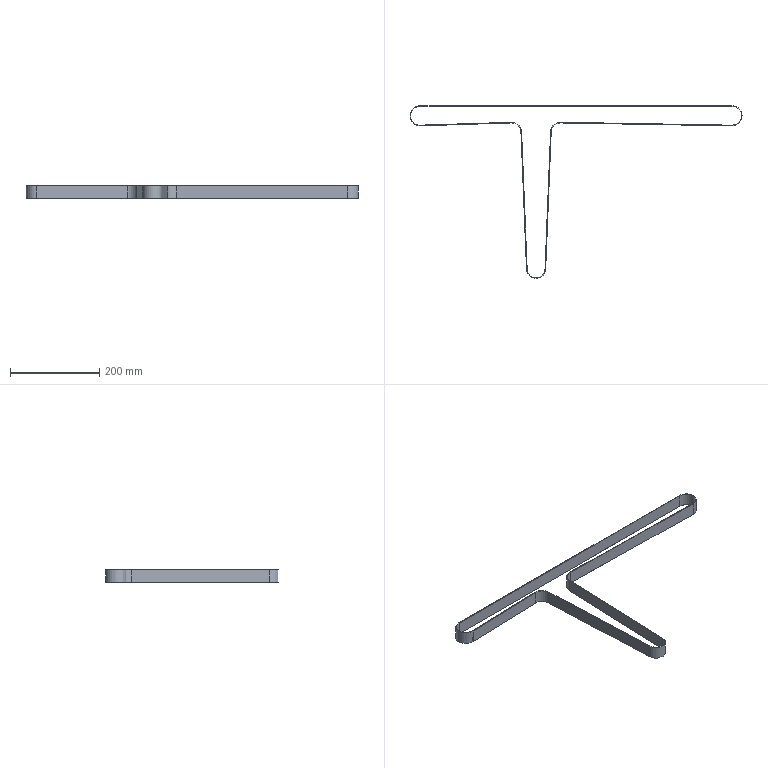Component | SolidWorks | Belt4-15^SW-111-1 | 1 solid | 24 faces | box 745 x 387 x 29 mm | volume 94519 mm3 | cylinder 12 | plane 12 | commonest cylinder face diameters 42 x5 45 x5 43 x1 40 x1
STEP:
#1=COLOUR_RGB('',0.7922,0.8196,0.9333);
#2=FILL_AREA_STYLE_COLOUR('',#1);
#3=FILL_AREA_STYLE('',(#2));
#4=SURFACE_STYLE_FILL_AREA(#3);
#5=SURFACE_SIDE_STYLE('',(#4));
#6=SURFACE_STYLE_USAGE(.BOTH.,#5);
#7=PRESENTATION_STYLE_ASSIGNMENT((#6));
#8=CARTESIAN_POINT('',(37.806,4.267,-1.437));
#9=VERTEX_POINT('',#8);
#10=CARTESIAN_POINT('',(36.98,5.094,-1.437));
#11=VERTEX_POINT('',#10);
#12=CARTESIAN_POINT('',(36.98,4.267,-1.437));
#13=DIRECTION('',(0.,0.,1.));
#14=DIRECTION('',(-1.,0.,0.));
#15=AXIS2_PLACEMENT_3D('',#12,#13,#14);
#16=CIRCLE('',#15,0.8268);
#17=EDGE_CURVE('',#9,#11,#16,.T.);
#18=ORIENTED_EDGE('',*,*,#17,.F.);
#19=CARTESIAN_POINT('',(37.806,4.267,-0.2953));
#20=VERTEX_POINT('',#19);
#21=CARTESIAN_POINT('',(37.806,4.267,-1.437));
#22=DIRECTION('',(0.,0.,1.));
#23=VECTOR('',#22,39.37);
#24=LINE('',#21,#23);
#25=EDGE_CURVE('',#9,#20,#24,.T.);
#26=ORIENTED_EDGE('',*,*,#25,.T.);
#27=CARTESIAN_POINT('',(36.98,5.094,-0.2953));
#28=VERTEX_POINT('',#27);
#29=CARTESIAN_POINT('',(36.98,4.267,-0.2953));
#30=DIRECTION('',(0.,0.,1.));
#31=DIRECTION('',(-1.,0.,0.));
#32=AXIS2_PLACEMENT_3D('',#29,#30,#31);
#33=CIRCLE('',#32,0.8268);
#34=EDGE_CURVE('',#20,#28,#33,.T.);
#35=ORIENTED_EDGE('',*,*,#34,.T.);
#36=CARTESIAN_POINT('',(36.98,5.094,-1.437));
#37=DIRECTION('',(0.,0.,1.));
#38=VECTOR('',#37,39.37);
#39=LINE('',#36,#38);
#40=EDGE_CURVE('',#11,#28,#39,.T.);
#41=ORIENTED_EDGE('',*,*,#40,.F.);
#42=EDGE_LOOP('',(#18,#26,#35,#41));
#43=FACE_OUTER_BOUND('',#42,.T.);
#44=CARTESIAN_POINT('',(36.98,4.267,-1.437));
#45=DIRECTION('',(0.,0.,1.));
#46=DIRECTION('',(1.,0.,0.));
#47=AXIS2_PLACEMENT_3D('',#44,#45,#46);
#48=CYLINDRICAL_SURFACE('',#47,0.8268);
#49=ADVANCED_FACE('',(#43),#48,.F.);
#50=CARTESIAN_POINT('',(36.965,3.381,-1.437));
#51=VERTEX_POINT('',#50);
#52=CARTESIAN_POINT('',(37.865,4.267,-1.437));
#53=VERTEX_POINT('',#52);
#54=CARTESIAN_POINT('',(36.98,4.267,-1.437));
#55=DIRECTION('',(0.,0.,1.));
#56=DIRECTION('',(-1.,0.,0.));
#57=AXIS2_PLACEMENT_3D('',#54,#55,#56);
#58=CIRCLE('',#57,0.8858);
#59=EDGE_CURVE('',#51,#53,#58,.T.);
#60=ORIENTED_EDGE('',*,*,#59,.T.);
#61=CARTESIAN_POINT('',(37.865,4.267,-0.2953));
#62=VERTEX_POINT('',#61);
#63=CARTESIAN_POINT('',(37.865,4.267,-1.437));
#64=DIRECTION('',(0.,0.,1.));
#65=VECTOR('',#64,39.37);
#66=LINE('',#63,#65);
#67=EDGE_CURVE('',#53,#62,#66,.T.);
#68=ORIENTED_EDGE('',*,*,#67,.T.);
#69=CARTESIAN_POINT('',(36.965,3.381,-0.2953));
#70=VERTEX_POINT('',#69);
#71=CARTESIAN_POINT('',(36.98,4.267,-0.2953));
#72=DIRECTION('',(0.,0.,1.));
#73=DIRECTION('',(-1.,0.,0.));
#74=AXIS2_PLACEMENT_3D('',#71,#72,#73);
#75=CIRCLE('',#74,0.8858);
#76=EDGE_CURVE('',#70,#62,#75,.T.);
#77=ORIENTED_EDGE('',*,*,#76,.F.);
#78=CARTESIAN_POINT('',(36.965,3.381,-1.437));
#79=DIRECTION('',(0.,0.,1.));
#80=VECTOR('',#79,39.37);
#81=LINE('',#78,#80);
#82=EDGE_CURVE('',#51,#70,#81,.T.);
#83=ORIENTED_EDGE('',*,*,#82,.F.);
#84=EDGE_LOOP('',(#60,#68,#77,#83));
#85=FACE_OUTER_BOUND('',#84,.T.);
#86=CARTESIAN_POINT('',(36.98,4.267,-1.437));
#87=DIRECTION('',(0.,0.,1.));
#88=DIRECTION('',(1.,0.,0.));
#89=AXIS2_PLACEMENT_3D('',#86,#87,#88);
#90=CYLINDRICAL_SURFACE('',#89,0.8858);
#91=ADVANCED_FACE('',(#85),#90,.T.);
#92=CARTESIAN_POINT('',(9.421,5.153,-0.2953));
#93=VERTEX_POINT('',#92);
#94=CARTESIAN_POINT('',(9.449,3.382,-0.2953));
#95=VERTEX_POINT('',#94);
#96=CARTESIAN_POINT('',(9.421,4.267,-0.2953));
#97=DIRECTION('',(0.,0.,1.));
#98=DIRECTION('',(-1.,0.,0.));
#99=AXIS2_PLACEMENT_3D('',#96,#97,#98);
#100=CIRCLE('',#99,0.8858);
#101=EDGE_CURVE('',#93,#95,#100,.T.);
#102=ORIENTED_EDGE('',*,*,#101,.F.);
#103=CARTESIAN_POINT('',(9.421,5.153,-1.437));
#104=VERTEX_POINT('',#103);
#105=CARTESIAN_POINT('',(9.421,5.153,-1.437));
#106=DIRECTION('',(0.,0.,1.));
#107=VECTOR('',#106,39.37);
#108=LINE('',#105,#107);
#109=EDGE_CURVE('',#104,#93,#108,.T.);
#110=ORIENTED_EDGE('',*,*,#109,.F.);
#111=CARTESIAN_POINT('',(9.449,3.382,-1.437));
#112=VERTEX_POINT('',#111);
#113=CARTESIAN_POINT('',(9.421,4.267,-1.437));
#114=DIRECTION('',(0.,0.,1.));
#115=DIRECTION('',(-1.,0.,0.));
#116=AXIS2_PLACEMENT_3D('',#113,#114,#115);
#117=CIRCLE('',#116,0.8858);
#118=EDGE_CURVE('',#104,#112,#117,.T.);
#119=ORIENTED_EDGE('',*,*,#118,.T.);
#120=CARTESIAN_POINT('',(9.449,3.382,-1.437));
#121=DIRECTION('',(0.,0.,1.));
#122=VECTOR('',#121,39.37);
#123=LINE('',#120,#122);
#124=EDGE_CURVE('',#112,#95,#123,.T.);
#125=ORIENTED_EDGE('',*,*,#124,.T.);
#126=EDGE_LOOP('',(#102,#110,#119,#125));
#127=FACE_OUTER_BOUND('',#126,.T.);
#128=CARTESIAN_POINT('',(9.421,4.267,-1.437));
#129=DIRECTION('',(0.,0.,1.));
#130=DIRECTION('',(1.,0.,0.));
#131=AXIS2_PLACEMENT_3D('',#128,#129,#130);
#132=CYLINDRICAL_SURFACE('',#131,0.8858);
#133=ADVANCED_FACE('',(#127),#132,.T.);
#134=CARTESIAN_POINT('',(36.98,5.153,-0.2953));
#135=VERTEX_POINT('',#134);
#136=CARTESIAN_POINT('',(9.421,5.153,-0.2953));
#137=DIRECTION('',(-1.,-0.,0.));
#138=VECTOR('',#137,39.37);
#139=LINE('',#136,#138);
#140=EDGE_CURVE('',#135,#93,#139,.T.);
#141=ORIENTED_EDGE('',*,*,#140,.F.);
#142=CARTESIAN_POINT('',(36.98,5.153,-1.437));
#143=VERTEX_POINT('',#142);
#144=CARTESIAN_POINT('',(36.98,5.153,-1.437));
#145=DIRECTION('',(0.,0.,1.));
#146=VECTOR('',#145,39.37);
#147=LINE('',#144,#146);
#148=EDGE_CURVE('',#143,#135,#147,.T.);
#149=ORIENTED_EDGE('',*,*,#148,.F.);
#150=CARTESIAN_POINT('',(9.421,5.153,-1.437));
#151=DIRECTION('',(-1.,-0.,0.));
#152=VECTOR('',#151,39.37);
#153=LINE('',#150,#152);
#154=EDGE_CURVE('',#143,#104,#153,.T.);
#155=ORIENTED_EDGE('',*,*,#154,.T.);
#156=ORIENTED_EDGE('',*,*,#109,.T.);
#157=EDGE_LOOP('',(#141,#149,#155,#156));
#158=FACE_OUTER_BOUND('',#157,.T.);
#159=CARTESIAN_POINT('',(9.421,5.153,-1.437));
#160=DIRECTION('',(-0.,1.,0.));
#161=DIRECTION('',(-1.,-0.,0.));
#162=AXIS2_PLACEMENT_3D('',#159,#160,#161);
#163=PLANE('',#162);
#164=ADVANCED_FACE('',(#158),#163,.T.);
#165=ORIENTED_EDGE('',*,*,#67,.F.);
#166=CARTESIAN_POINT('',(36.98,4.267,-1.437));
#167=DIRECTION('',(0.,0.,1.));
#168=DIRECTION('',(-1.,0.,0.));
#169=AXIS2_PLACEMENT_3D('',#166,#167,#168);
#170=CIRCLE('',#169,0.8858);
#171=EDGE_CURVE('',#53,#143,#170,.T.);
#172=ORIENTED_EDGE('',*,*,#171,.T.);
#173=ORIENTED_EDGE('',*,*,#148,.T.);
#174=CARTESIAN_POINT('',(36.98,4.267,-0.2953));
#175=DIRECTION('',(0.,0.,1.));
#176=DIRECTION('',(-1.,0.,0.));
#177=AXIS2_PLACEMENT_3D('',#174,#175,#176);
#178=CIRCLE('',#177,0.8858);
#179=EDGE_CURVE('',#62,#135,#178,.T.);
#180=ORIENTED_EDGE('',*,*,#179,.F.);
#181=EDGE_LOOP('',(#165,#172,#173,#180));
#182=FACE_OUTER_BOUND('',#181,.T.);
#183=CARTESIAN_POINT('',(36.98,4.267,-1.437));
#184=DIRECTION('',(0.,0.,1.));
#185=DIRECTION('',(1.,0.,0.));
#186=AXIS2_PLACEMENT_3D('',#183,#184,#185);
#187=CYLINDRICAL_SURFACE('',#186,0.8858);
#188=ADVANCED_FACE('',(#182),#187,.T.);
#189=CARTESIAN_POINT('',(21.856,3.637,-0.2953));
#190=VERTEX_POINT('',#189);
#191=CARTESIAN_POINT('',(9.414,3.848,-0.2953));
#192=DIRECTION('',(0.9999,-0.01692,0.));
#193=VECTOR('',#192,39.37);
#194=LINE('',#191,#193);
#195=EDGE_CURVE('',#190,#70,#194,.T.);
#196=ORIENTED_EDGE('',*,*,#195,.F.);
#197=CARTESIAN_POINT('',(21.856,3.637,-1.437));
#198=VERTEX_POINT('',#197);
#199=CARTESIAN_POINT('',(21.856,3.637,-1.437));
#200=DIRECTION('',(0.,0.,1.));
#201=VECTOR('',#200,39.37);
#202=LINE('',#199,#201);
#203=EDGE_CURVE('',#198,#190,#202,.T.);
#204=ORIENTED_EDGE('',*,*,#203,.F.);
#205=CARTESIAN_POINT('',(9.414,3.848,-1.437));
#206=DIRECTION('',(0.9999,-0.01692,0.));
#207=VECTOR('',#206,39.37);
#208=LINE('',#205,#207);
#209=EDGE_CURVE('',#198,#51,#208,.T.);
#210=ORIENTED_EDGE('',*,*,#209,.T.);
#211=ORIENTED_EDGE('',*,*,#82,.T.);
#212=EDGE_LOOP('',(#196,#204,#210,#211));
#213=FACE_OUTER_BOUND('',#212,.T.);
#214=CARTESIAN_POINT('',(9.414,3.848,-1.437));
#215=DIRECTION('',(-0.01692,-0.9999,0.));
#216=DIRECTION('',(0.9999,-0.01692,0.));
#217=AXIS2_PLACEMENT_3D('',#214,#215,#216);
#218=PLANE('',#217);
#219=ADVANCED_FACE('',(#213),#218,.T.);
#220=CARTESIAN_POINT('',(21.016,2.844,-0.2953));
#221=VERTEX_POINT('',#220);
#222=CARTESIAN_POINT('',(21.842,2.81,-0.2953));
#223=DIRECTION('',(0.,0.,-1.));
#224=DIRECTION('',(-1.,0.,0.));
#225=AXIS2_PLACEMENT_3D('',#222,#223,#224);
#226=CIRCLE('',#225,0.8268);
#227=EDGE_CURVE('',#221,#190,#226,.T.);
#228=ORIENTED_EDGE('',*,*,#227,.F.);
#229=CARTESIAN_POINT('',(21.016,2.844,-1.437));
#230=VERTEX_POINT('',#229);
#231=CARTESIAN_POINT('',(21.016,2.844,-1.437));
#232=DIRECTION('',(0.,0.,1.));
#233=VECTOR('',#232,39.37);
#234=LINE('',#231,#233);
#235=EDGE_CURVE('',#230,#221,#234,.T.);
#236=ORIENTED_EDGE('',*,*,#235,.F.);
#237=CARTESIAN_POINT('',(21.842,2.81,-1.437));
#238=DIRECTION('',(0.,0.,-1.));
#239=DIRECTION('',(-1.,0.,0.));
#240=AXIS2_PLACEMENT_3D('',#237,#238,#239);
#241=CIRCLE('',#240,0.8268);
#242=EDGE_CURVE('',#230,#198,#241,.T.);
#243=ORIENTED_EDGE('',*,*,#242,.T.);
#244=ORIENTED_EDGE('',*,*,#203,.T.);
#245=EDGE_LOOP('',(#228,#236,#243,#244));
#246=FACE_OUTER_BOUND('',#245,.T.);
#247=CARTESIAN_POINT('',(21.842,2.81,-1.437));
#248=DIRECTION('',(0.,0.,1.));
#249=DIRECTION('',(1.,0.,0.));
#250=AXIS2_PLACEMENT_3D('',#247,#248,#249);
#251=CYLINDRICAL_SURFACE('',#250,0.8268);
#252=ADVANCED_FACE('',(#246),#251,.F.);
#253=CARTESIAN_POINT('',(20.522,-9.271,-0.2953));
#254=VERTEX_POINT('',#253);
#255=CARTESIAN_POINT('',(21.054,3.793,-0.2953));
#256=DIRECTION('',(0.0407,0.9992,0.));
#257=VECTOR('',#256,39.37);
#258=LINE('',#255,#257);
#259=EDGE_CURVE('',#254,#221,#258,.T.);
#260=ORIENTED_EDGE('',*,*,#259,.F.);
#261=CARTESIAN_POINT('',(20.522,-9.271,-1.437));
#262=VERTEX_POINT('',#261);
#263=CARTESIAN_POINT('',(20.522,-9.271,-1.437));
#264=DIRECTION('',(0.,0.,1.));
#265=VECTOR('',#264,39.37);
#266=LINE('',#263,#265);
#267=EDGE_CURVE('',#262,#254,#266,.T.);
#268=ORIENTED_EDGE('',*,*,#267,.F.);
#269=CARTESIAN_POINT('',(21.054,3.793,-1.437));
#270=DIRECTION('',(0.0407,0.9992,0.));
#271=VECTOR('',#270,39.37);
#272=LINE('',#269,#271);
#273=EDGE_CURVE('',#262,#230,#272,.T.);
#274=ORIENTED_EDGE('',*,*,#273,.T.);
#275=ORIENTED_EDGE('',*,*,#235,.T.);
#276=EDGE_LOOP('',(#260,#268,#274,#275));
#277=FACE_OUTER_BOUND('',#276,.T.);
#278=CARTESIAN_POINT('',(21.054,3.793,-1.437));
#279=DIRECTION('',(0.9992,-0.0407,0.));
#280=DIRECTION('',(0.0407,0.9992,0.));
#281=AXIS2_PLACEMENT_3D('',#278,#279,#280);
#282=PLANE('',#281);
#283=ADVANCED_FACE('',(#277),#282,.T.);
#284=CARTESIAN_POINT('',(18.831,-9.271,-0.2953));
#285=VERTEX_POINT('',#284);
#286=CARTESIAN_POINT('',(19.677,-9.237,-0.2953));
#287=DIRECTION('',(0.,0.,1.));
#288=DIRECTION('',(-1.,0.,0.));
#289=AXIS2_PLACEMENT_3D('',#286,#287,#288);
#290=CIRCLE('',#289,0.8465);
#291=EDGE_CURVE('',#285,#254,#290,.T.);
#292=ORIENTED_EDGE('',*,*,#291,.F.);
#293=CARTESIAN_POINT('',(18.831,-9.271,-1.437));
#294=VERTEX_POINT('',#293);
#295=CARTESIAN_POINT('',(18.831,-9.271,-1.437));
#296=DIRECTION('',(0.,0.,1.));
#297=VECTOR('',#296,39.37);
#298=LINE('',#295,#297);
#299=EDGE_CURVE('',#294,#285,#298,.T.);
#300=ORIENTED_EDGE('',*,*,#299,.F.);
#301=CARTESIAN_POINT('',(19.677,-9.237,-1.437));
#302=DIRECTION('',(0.,0.,1.));
#303=DIRECTION('',(-1.,0.,0.));
#304=AXIS2_PLACEMENT_3D('',#301,#302,#303);
#305=CIRCLE('',#304,0.8465);
#306=EDGE_CURVE('',#294,#262,#305,.T.);
#307=ORIENTED_EDGE('',*,*,#306,.T.);
#308=ORIENTED_EDGE('',*,*,#267,.T.);
#309=EDGE_LOOP('',(#292,#300,#307,#308));
#310=FACE_OUTER_BOUND('',#309,.T.);
#311=CARTESIAN_POINT('',(19.677,-9.237,-1.437));
#312=DIRECTION('',(0.,0.,1.));
#313=DIRECTION('',(1.,0.,0.));
#314=AXIS2_PLACEMENT_3D('',#311,#312,#313);
#315=CYLINDRICAL_SURFACE('',#314,0.8465);
#316=ADVANCED_FACE('',(#310),#315,.T.);
#317=CARTESIAN_POINT('',(18.337,2.844,-0.2953));
#318=VERTEX_POINT('',#317);
#319=CARTESIAN_POINT('',(18.265,4.627,-0.2953));
#320=DIRECTION('',(0.0407,-0.9992,0.));
#321=VECTOR('',#320,39.37);
#322=LINE('',#319,#321);
#323=EDGE_CURVE('',#318,#285,#322,.T.);
#324=ORIENTED_EDGE('',*,*,#323,.F.);
#325=CARTESIAN_POINT('',(18.337,2.844,-1.437));
#326=VERTEX_POINT('',#325);
#327=CARTESIAN_POINT('',(18.337,2.844,-1.437));
#328=DIRECTION('',(0.,0.,1.));
#329=VECTOR('',#328,39.37);
#330=LINE('',#327,#329);
#331=EDGE_CURVE('',#326,#318,#330,.T.);
#332=ORIENTED_EDGE('',*,*,#331,.F.);
#333=CARTESIAN_POINT('',(18.265,4.627,-1.437));
#334=DIRECTION('',(0.0407,-0.9992,0.));
#335=VECTOR('',#334,39.37);
#336=LINE('',#333,#335);
#337=EDGE_CURVE('',#326,#294,#336,.T.);
#338=ORIENTED_EDGE('',*,*,#337,.T.);
#339=ORIENTED_EDGE('',*,*,#299,.T.);
#340=EDGE_LOOP('',(#324,#332,#338,#339));
#341=FACE_OUTER_BOUND('',#340,.T.);
#342=CARTESIAN_POINT('',(18.265,4.627,-1.437));
#343=DIRECTION('',(-0.9992,-0.0407,0.));
#344=DIRECTION('',(0.0407,-0.9992,0.));
#345=AXIS2_PLACEMENT_3D('',#342,#343,#344);
#346=PLANE('',#345);
#347=ADVANCED_FACE('',(#341),#346,.T.);
#348=CARTESIAN_POINT('',(17.485,3.637,-0.2953));
#349=VERTEX_POINT('',#348);
#350=CARTESIAN_POINT('',(17.511,2.81,-0.2953));
#351=DIRECTION('',(0.,0.,-1.));
#352=DIRECTION('',(-1.,0.,0.));
#353=AXIS2_PLACEMENT_3D('',#350,#351,#352);
#354=CIRCLE('',#353,0.8268);
#355=EDGE_CURVE('',#349,#318,#354,.T.);
#356=ORIENTED_EDGE('',*,*,#355,.F.);
#357=CARTESIAN_POINT('',(17.485,3.637,-1.437));
#358=VERTEX_POINT('',#357);
#359=CARTESIAN_POINT('',(17.485,3.637,-1.437));
#360=DIRECTION('',(0.,0.,1.));
#361=VECTOR('',#360,39.37);
#362=LINE('',#359,#361);
#363=EDGE_CURVE('',#358,#349,#362,.T.);
#364=ORIENTED_EDGE('',*,*,#363,.F.);
#365=CARTESIAN_POINT('',(17.511,2.81,-1.437));
#366=DIRECTION('',(0.,0.,-1.));
#367=DIRECTION('',(-1.,0.,0.));
#368=AXIS2_PLACEMENT_3D('',#365,#366,#367);
#369=CIRCLE('',#368,0.8268);
#370=EDGE_CURVE('',#358,#326,#369,.T.);
#371=ORIENTED_EDGE('',*,*,#370,.T.);
#372=ORIENTED_EDGE('',*,*,#331,.T.);
#373=EDGE_LOOP('',(#356,#364,#371,#372));
#374=FACE_OUTER_BOUND('',#373,.T.);
#375=CARTESIAN_POINT('',(17.511,2.81,-1.437));
#376=DIRECTION('',(0.,0.,1.));
#377=DIRECTION('',(1.,0.,0.));
#378=AXIS2_PLACEMENT_3D('',#375,#376,#377);
#379=CYLINDRICAL_SURFACE('',#378,0.8268);
#380=ADVANCED_FACE('',(#374),#379,.F.);
#381=CARTESIAN_POINT('',(9.449,3.382,-0.2953));
#382=DIRECTION('',(0.9995,0.03172,0.));
#383=VECTOR('',#382,39.37);
#384=LINE('',#381,#383);
#385=EDGE_CURVE('',#95,#349,#384,.T.);
#386=ORIENTED_EDGE('',*,*,#385,.F.);
#387=ORIENTED_EDGE('',*,*,#124,.F.);
#388=CARTESIAN_POINT('',(9.449,3.382,-1.437));
#389=DIRECTION('',(0.9995,0.03172,0.));
#390=VECTOR('',#389,39.37);
#391=LINE('',#388,#390);
#392=EDGE_CURVE('',#112,#358,#391,.T.);
#393=ORIENTED_EDGE('',*,*,#392,.T.);
#394=ORIENTED_EDGE('',*,*,#363,.T.);
#395=EDGE_LOOP('',(#386,#387,#393,#394));
#396=FACE_OUTER_BOUND('',#395,.T.);
#397=CARTESIAN_POINT('',(9.449,3.382,-1.437));
#398=DIRECTION('',(0.03172,-0.9995,0.));
#399=DIRECTION('',(0.9995,0.03172,0.));
#400=AXIS2_PLACEMENT_3D('',#397,#398,#399);
#401=PLANE('',#400);
#402=ADVANCED_FACE('',(#396),#401,.T.);
#403=CARTESIAN_POINT('',(9.421,5.094,-1.437));
#404=VERTEX_POINT('',#403);
#405=CARTESIAN_POINT('',(9.447,3.441,-1.437));
#406=VERTEX_POINT('',#405);
#407=CARTESIAN_POINT('',(9.421,4.267,-1.437));
#408=DIRECTION('',(0.,0.,1.));
#409=DIRECTION('',(-1.,0.,0.));
#410=AXIS2_PLACEMENT_3D('',#407,#408,#409);
#411=CIRCLE('',#410,0.8268);
#412=EDGE_CURVE('',#404,#406,#411,.T.);
#413=ORIENTED_EDGE('',*,*,#412,.T.);
#414=CARTESIAN_POINT('',(17.483,3.696,-1.437));
#415=VERTEX_POINT('',#414);
#416=CARTESIAN_POINT('',(17.483,3.696,-1.437));
#417=DIRECTION('',(0.9995,0.03172,0.));
#418=VECTOR('',#417,39.37);
#419=LINE('',#416,#418);
#420=EDGE_CURVE('',#406,#415,#419,.T.);
#421=ORIENTED_EDGE('',*,*,#420,.T.);
#422=CARTESIAN_POINT('',(18.396,2.846,-1.437));
#423=VERTEX_POINT('',#422);
#424=CARTESIAN_POINT('',(17.511,2.81,-1.437));
#425=DIRECTION('',(0.,0.,-1.));
#426=DIRECTION('',(1.,0.,0.));
#427=AXIS2_PLACEMENT_3D('',#424,#425,#426);
#428=CIRCLE('',#427,0.8858);
#429=EDGE_CURVE('',#415,#423,#428,.T.);
#430=ORIENTED_EDGE('',*,*,#429,.T.);
#431=CARTESIAN_POINT('',(18.89,-9.269,-1.437));
#432=VERTEX_POINT('',#431);
#433=CARTESIAN_POINT('',(18.89,-9.269,-1.437));
#434=DIRECTION('',(0.0407,-0.9992,0.));
#435=VECTOR('',#434,39.37);
#436=LINE('',#433,#435);
#437=EDGE_CURVE('',#423,#432,#436,.T.);
#438=ORIENTED_EDGE('',*,*,#437,.T.);
#439=CARTESIAN_POINT('',(20.463,-9.269,-1.437));
#440=VERTEX_POINT('',#439);
#441=CARTESIAN_POINT('',(19.677,-9.237,-1.437));
#442=DIRECTION('',(0.,0.,1.));
#443=DIRECTION('',(-1.,0.,0.));
#444=AXIS2_PLACEMENT_3D('',#441,#442,#443);
#445=CIRCLE('',#444,0.7874);
#446=EDGE_CURVE('',#432,#440,#445,.T.);
#447=ORIENTED_EDGE('',*,*,#446,.T.);
#448=CARTESIAN_POINT('',(20.957,2.846,-1.437));
#449=VERTEX_POINT('',#448);
#450=CARTESIAN_POINT('',(20.957,2.846,-1.437));
#451=DIRECTION('',(0.0407,0.9992,0.));
#452=VECTOR('',#451,39.37);
#453=LINE('',#450,#452);
#454=EDGE_CURVE('',#440,#449,#453,.T.);
#455=ORIENTED_EDGE('',*,*,#454,.T.);
#456=CARTESIAN_POINT('',(21.857,3.696,-1.437));
#457=VERTEX_POINT('',#456);
#458=CARTESIAN_POINT('',(21.842,2.81,-1.437));
#459=DIRECTION('',(0.,0.,-1.));
#460=DIRECTION('',(1.,0.,0.));
#461=AXIS2_PLACEMENT_3D('',#458,#459,#460);
#462=CIRCLE('',#461,0.8858);
#463=EDGE_CURVE('',#449,#457,#462,.T.);
#464=ORIENTED_EDGE('',*,*,#463,.T.);
#465=CARTESIAN_POINT('',(36.966,3.44,-1.437));
#466=VERTEX_POINT('',#465);
#467=CARTESIAN_POINT('',(36.966,3.44,-1.437));
#468=DIRECTION('',(0.9999,-0.01692,0.));
#469=VECTOR('',#468,39.37);
#470=LINE('',#467,#469);
#471=EDGE_CURVE('',#457,#466,#470,.T.);
#472=ORIENTED_EDGE('',*,*,#471,.T.);
#473=CARTESIAN_POINT('',(36.98,4.267,-1.437));
#474=DIRECTION('',(0.,0.,1.));
#475=DIRECTION('',(-1.,0.,0.));
#476=AXIS2_PLACEMENT_3D('',#473,#474,#475);
#477=CIRCLE('',#476,0.8268);
#478=EDGE_CURVE('',#466,#9,#477,.T.);
#479=ORIENTED_EDGE('',*,*,#478,.T.);
#480=ORIENTED_EDGE('',*,*,#17,.T.);
#481=CARTESIAN_POINT('',(9.421,5.094,-1.437));
#482=DIRECTION('',(-1.,-0.,0.));
#483=VECTOR('',#482,39.37);
#484=LINE('',#481,#483);
#485=EDGE_CURVE('',#11,#404,#484,.T.);
#486=ORIENTED_EDGE('',*,*,#485,.T.);
#487=EDGE_LOOP('',(#413,#421,#430,#438,#447,#455,#464,#472,#479,#480,#486));
#488=FACE_BOUND('',#487,.T.);
#489=ORIENTED_EDGE('',*,*,#118,.F.);
#490=ORIENTED_EDGE('',*,*,#154,.F.);
#491=ORIENTED_EDGE('',*,*,#171,.F.);
#492=ORIENTED_EDGE('',*,*,#59,.F.);
#493=ORIENTED_EDGE('',*,*,#209,.F.);
#494=ORIENTED_EDGE('',*,*,#242,.F.);
#495=ORIENTED_EDGE('',*,*,#273,.F.);
#496=ORIENTED_EDGE('',*,*,#306,.F.);
#497=ORIENTED_EDGE('',*,*,#337,.F.);
#498=ORIENTED_EDGE('',*,*,#370,.F.);
#499=ORIENTED_EDGE('',*,*,#392,.F.);
#500=EDGE_LOOP('',(#489,#490,#491,#492,#493,#494,#495,#496,#497,#498,#499));
#501=FACE_OUTER_BOUND('',#500,.T.);
#502=CARTESIAN_POINT('',(9.421,4.267,-1.437));
#503=DIRECTION('',(0.,0.,-1.));
#504=DIRECTION('',(-1.,0.,0.));
#505=AXIS2_PLACEMENT_3D('',#502,#503,#504);
#506=PLANE('',#505);
#507=ADVANCED_FACE('',(#488,#501),#506,.T.);
#508=CARTESIAN_POINT('',(9.447,3.441,-0.2953));
#509=VERTEX_POINT('',#508);
#510=CARTESIAN_POINT('',(17.483,3.696,-0.2953));
#511=VERTEX_POINT('',#510);
#512=CARTESIAN_POINT('',(17.483,3.696,-0.2953));
#513=DIRECTION('',(0.9995,0.03172,0.));
#514=VECTOR('',#513,39.37);
#515=LINE('',#512,#514);
#516=EDGE_CURVE('',#509,#511,#515,.T.);
#517=ORIENTED_EDGE('',*,*,#516,.F.);
#518=CARTESIAN_POINT('',(9.421,5.094,-0.2953));
#519=VERTEX_POINT('',#518);
#520=CARTESIAN_POINT('',(9.421,4.267,-0.2953));
#521=DIRECTION('',(0.,0.,1.));
#522=DIRECTION('',(-1.,0.,0.));
#523=AXIS2_PLACEMENT_3D('',#520,#521,#522);
#524=CIRCLE('',#523,0.8268);
#525=EDGE_CURVE('',#519,#509,#524,.T.);
#526=ORIENTED_EDGE('',*,*,#525,.F.);
#527=CARTESIAN_POINT('',(9.421,5.094,-0.2953));
#528=DIRECTION('',(-1.,-0.,0.));
#529=VECTOR('',#528,39.37);
#530=LINE('',#527,#529);
#531=EDGE_CURVE('',#28,#519,#530,.T.);
#532=ORIENTED_EDGE('',*,*,#531,.F.);
#533=ORIENTED_EDGE('',*,*,#34,.F.);
#534=CARTESIAN_POINT('',(36.966,3.44,-0.2953));
#535=VERTEX_POINT('',#534);
#536=CARTESIAN_POINT('',(36.98,4.267,-0.2953));
#537=DIRECTION('',(0.,0.,1.));
#538=DIRECTION('',(-1.,0.,0.));
#539=AXIS2_PLACEMENT_3D('',#536,#537,#538);
#540=CIRCLE('',#539,0.8268);
#541=EDGE_CURVE('',#535,#20,#540,.T.);
#542=ORIENTED_EDGE('',*,*,#541,.F.);
#543=CARTESIAN_POINT('',(21.857,3.696,-0.2953));
#544=VERTEX_POINT('',#543);
#545=CARTESIAN_POINT('',(36.966,3.44,-0.2953));
#546=DIRECTION('',(0.9999,-0.01692,0.));
#547=VECTOR('',#546,39.37);
#548=LINE('',#545,#547);
#549=EDGE_CURVE('',#544,#535,#548,.T.);
#550=ORIENTED_EDGE('',*,*,#549,.F.);
#551=CARTESIAN_POINT('',(20.957,2.846,-0.2953));
#552=VERTEX_POINT('',#551);
#553=CARTESIAN_POINT('',(21.842,2.81,-0.2953));
#554=DIRECTION('',(0.,0.,-1.));
#555=DIRECTION('',(1.,0.,0.));
#556=AXIS2_PLACEMENT_3D('',#553,#554,#555);
#557=CIRCLE('',#556,0.8858);
#558=EDGE_CURVE('',#552,#544,#557,.T.);
#559=ORIENTED_EDGE('',*,*,#558,.F.);
#560=CARTESIAN_POINT('',(20.463,-9.269,-0.2953));
#561=VERTEX_POINT('',#560);
#562=CARTESIAN_POINT('',(20.957,2.846,-0.2953));
#563=DIRECTION('',(0.0407,0.9992,0.));
#564=VECTOR('',#563,39.37);
#565=LINE('',#562,#564);
#566=EDGE_CURVE('',#561,#552,#565,.T.);
#567=ORIENTED_EDGE('',*,*,#566,.F.);
#568=CARTESIAN_POINT('',(18.89,-9.269,-0.2953));
#569=VERTEX_POINT('',#568);
#570=CARTESIAN_POINT('',(19.677,-9.237,-0.2953));
#571=DIRECTION('',(0.,0.,1.));
#572=DIRECTION('',(-1.,0.,0.));
#573=AXIS2_PLACEMENT_3D('',#570,#571,#572);
#574=CIRCLE('',#573,0.7874);
#575=EDGE_CURVE('',#569,#561,#574,.T.);
#576=ORIENTED_EDGE('',*,*,#575,.F.);
#577=CARTESIAN_POINT('',(18.396,2.846,-0.2953));
#578=VERTEX_POINT('',#577);
#579=CARTESIAN_POINT('',(18.89,-9.269,-0.2953));
#580=DIRECTION('',(0.0407,-0.9992,0.));
#581=VECTOR('',#580,39.37);
#582=LINE('',#579,#581);
#583=EDGE_CURVE('',#578,#569,#582,.T.);
#584=ORIENTED_EDGE('',*,*,#583,.F.);
#585=CARTESIAN_POINT('',(17.511,2.81,-0.2953));
#586=DIRECTION('',(0.,0.,-1.));
#587=DIRECTION('',(1.,0.,0.));
#588=AXIS2_PLACEMENT_3D('',#585,#586,#587);
#589=CIRCLE('',#588,0.8858);
#590=EDGE_CURVE('',#511,#578,#589,.T.);
#591=ORIENTED_EDGE('',*,*,#590,.F.);
#592=EDGE_LOOP('',(#517,#526,#532,#533,#542,#550,#559,#567,#576,#584,#591));
#593=FACE_BOUND('',#592,.T.);
#594=ORIENTED_EDGE('',*,*,#101,.T.);
#595=ORIENTED_EDGE('',*,*,#385,.T.);
#596=ORIENTED_EDGE('',*,*,#355,.T.);
#597=ORIENTED_EDGE('',*,*,#323,.T.);
#598=ORIENTED_EDGE('',*,*,#291,.T.);
#599=ORIENTED_EDGE('',*,*,#259,.T.);
#600=ORIENTED_EDGE('',*,*,#227,.T.);
#601=ORIENTED_EDGE('',*,*,#195,.T.);
#602=ORIENTED_EDGE('',*,*,#76,.T.);
#603=ORIENTED_EDGE('',*,*,#179,.T.);
#604=ORIENTED_EDGE('',*,*,#140,.T.);
#605=EDGE_LOOP('',(#594,#595,#596,#597,#598,#599,#600,#601,#602,#603,#604));
#606=FACE_OUTER_BOUND('',#605,.T.);
#607=CARTESIAN_POINT('',(9.421,4.267,-0.2953));
#608=DIRECTION('',(0.,0.,-1.));
#609=DIRECTION('',(-1.,0.,0.));
#610=AXIS2_PLACEMENT_3D('',#607,#608,#609);
#611=PLANE('',#610);
#612=ADVANCED_FACE('',(#593,#606),#611,.F.);
#613=ORIENTED_EDGE('',*,*,#525,.T.);
#614=CARTESIAN_POINT('',(9.447,3.441,-1.437));
#615=DIRECTION('',(0.,0.,1.));
#616=VECTOR('',#615,39.37);
#617=LINE('',#614,#616);
#618=EDGE_CURVE('',#406,#509,#617,.T.);
#619=ORIENTED_EDGE('',*,*,#618,.F.);
#620=ORIENTED_EDGE('',*,*,#412,.F.);
#621=CARTESIAN_POINT('',(9.421,5.094,-1.437));
#622=DIRECTION('',(0.,0.,1.));
#623=VECTOR('',#622,39.37);
#624=LINE('',#621,#623);
#625=EDGE_CURVE('',#404,#519,#624,.T.);
#626=ORIENTED_EDGE('',*,*,#625,.T.);
#627=EDGE_LOOP('',(#613,#619,#620,#626));
#628=FACE_OUTER_BOUND('',#627,.T.);
#629=CARTESIAN_POINT('',(9.421,4.267,-1.437));
#630=DIRECTION('',(0.,0.,1.));
#631=DIRECTION('',(1.,0.,0.));
#632=AXIS2_PLACEMENT_3D('',#629,#630,#631);
#633=CYLINDRICAL_SURFACE('',#632,0.8268);
#634=ADVANCED_FACE('',(#628),#633,.F.);
#635=ORIENTED_EDGE('',*,*,#531,.T.);
#636=ORIENTED_EDGE('',*,*,#625,.F.);
#637=ORIENTED_EDGE('',*,*,#485,.F.);
#638=ORIENTED_EDGE('',*,*,#40,.T.);
#639=EDGE_LOOP('',(#635,#636,#637,#638));
#640=FACE_OUTER_BOUND('',#639,.T.);
#641=CARTESIAN_POINT('',(9.421,5.094,-1.437));
#642=DIRECTION('',(-0.,1.,0.));
#643=DIRECTION('',(-1.,-0.,0.));
#644=AXIS2_PLACEMENT_3D('',#641,#642,#643);
#645=PLANE('',#644);
#646=ADVANCED_FACE('',(#640),#645,.F.);
#647=ORIENTED_EDGE('',*,*,#25,.F.);
#648=ORIENTED_EDGE('',*,*,#478,.F.);
#649=CARTESIAN_POINT('',(36.966,3.44,-1.437));
#650=DIRECTION('',(0.,0.,1.));
#651=VECTOR('',#650,39.37);
#652=LINE('',#649,#651);
#653=EDGE_CURVE('',#466,#535,#652,.T.);
#654=ORIENTED_EDGE('',*,*,#653,.T.);
#655=ORIENTED_EDGE('',*,*,#541,.T.);
#656=EDGE_LOOP('',(#647,#648,#654,#655));
#657=FACE_OUTER_BOUND('',#656,.T.);
#658=CARTESIAN_POINT('',(36.98,4.267,-1.437));
#659=DIRECTION('',(0.,0.,1.));
#660=DIRECTION('',(1.,0.,0.));
#661=AXIS2_PLACEMENT_3D('',#658,#659,#660);
#662=CYLINDRICAL_SURFACE('',#661,0.8268);
#663=ADVANCED_FACE('',(#657),#662,.F.);
#664=ORIENTED_EDGE('',*,*,#549,.T.);
#665=ORIENTED_EDGE('',*,*,#653,.F.);
#666=ORIENTED_EDGE('',*,*,#471,.F.);
#667=CARTESIAN_POINT('',(21.857,3.696,-1.437));
#668=DIRECTION('',(0.,0.,1.));
#669=VECTOR('',#668,39.37);
#670=LINE('',#667,#669);
#671=EDGE_CURVE('',#457,#544,#670,.T.);
#672=ORIENTED_EDGE('',*,*,#671,.T.);
#673=EDGE_LOOP('',(#664,#665,#666,#672));
#674=FACE_OUTER_BOUND('',#673,.T.);
#675=CARTESIAN_POINT('',(36.966,3.44,-1.437));
#676=DIRECTION('',(-0.01692,-0.9999,0.));
#677=DIRECTION('',(0.9999,-0.01692,0.));
#678=AXIS2_PLACEMENT_3D('',#675,#676,#677);
#679=PLANE('',#678);
#680=ADVANCED_FACE('',(#674),#679,.F.);
#681=ORIENTED_EDGE('',*,*,#558,.T.);
#682=ORIENTED_EDGE('',*,*,#671,.F.);
#683=ORIENTED_EDGE('',*,*,#463,.F.);
#684=CARTESIAN_POINT('',(20.957,2.846,-1.437));
#685=DIRECTION('',(0.,0.,1.));
#686=VECTOR('',#685,39.37);
#687=LINE('',#684,#686);
#688=EDGE_CURVE('',#449,#552,#687,.T.);
#689=ORIENTED_EDGE('',*,*,#688,.T.);
#690=EDGE_LOOP('',(#681,#682,#683,#689));
#691=FACE_OUTER_BOUND('',#690,.T.);
#692=CARTESIAN_POINT('',(21.842,2.81,-1.437));
#693=DIRECTION('',(0.,0.,1.));
#694=DIRECTION('',(1.,0.,0.));
#695=AXIS2_PLACEMENT_3D('',#692,#693,#694);
#696=CYLINDRICAL_SURFACE('',#695,0.8858);
#697=ADVANCED_FACE('',(#691),#696,.T.);
#698=ORIENTED_EDGE('',*,*,#566,.T.);
#699=ORIENTED_EDGE('',*,*,#688,.F.);
#700=ORIENTED_EDGE('',*,*,#454,.F.);
#701=CARTESIAN_POINT('',(20.463,-9.269,-1.437));
#702=DIRECTION('',(0.,0.,1.));
#703=VECTOR('',#702,39.37);
#704=LINE('',#701,#703);
#705=EDGE_CURVE('',#440,#561,#704,.T.);
#706=ORIENTED_EDGE('',*,*,#705,.T.);
#707=EDGE_LOOP('',(#698,#699,#700,#706));
#708=FACE_OUTER_BOUND('',#707,.T.);
#709=CARTESIAN_POINT('',(20.957,2.846,-1.437));
#710=DIRECTION('',(0.9992,-0.0407,0.));
#711=DIRECTION('',(0.0407,0.9992,0.));
#712=AXIS2_PLACEMENT_3D('',#709,#710,#711);
#713=PLANE('',#712);
#714=ADVANCED_FACE('',(#708),#713,.F.);
#715=ORIENTED_EDGE('',*,*,#575,.T.);
#716=ORIENTED_EDGE('',*,*,#705,.F.);
#717=ORIENTED_EDGE('',*,*,#446,.F.);
#718=CARTESIAN_POINT('',(18.89,-9.269,-1.437));
#719=DIRECTION('',(0.,0.,1.));
#720=VECTOR('',#719,39.37);
#721=LINE('',#718,#720);
#722=EDGE_CURVE('',#432,#569,#721,.T.);
#723=ORIENTED_EDGE('',*,*,#722,.T.);
#724=EDGE_LOOP('',(#715,#716,#717,#723));
#725=FACE_OUTER_BOUND('',#724,.T.);
#726=CARTESIAN_POINT('',(19.677,-9.237,-1.437));
#727=DIRECTION('',(0.,0.,1.));
#728=DIRECTION('',(1.,0.,0.));
#729=AXIS2_PLACEMENT_3D('',#726,#727,#728);
#730=CYLINDRICAL_SURFACE('',#729,0.7874);
#731=ADVANCED_FACE('',(#725),#730,.F.);
#732=ORIENTED_EDGE('',*,*,#583,.T.);
#733=ORIENTED_EDGE('',*,*,#722,.F.);
#734=ORIENTED_EDGE('',*,*,#437,.F.);
#735=CARTESIAN_POINT('',(18.396,2.846,-1.437));
#736=DIRECTION('',(0.,0.,1.));
#737=VECTOR('',#736,39.37);
#738=LINE('',#735,#737);
#739=EDGE_CURVE('',#423,#578,#738,.T.);
#740=ORIENTED_EDGE('',*,*,#739,.T.);
#741=EDGE_LOOP('',(#732,#733,#734,#740));
#742=FACE_OUTER_BOUND('',#741,.T.);
#743=CARTESIAN_POINT('',(18.89,-9.269,-1.437));
#744=DIRECTION('',(-0.9992,-0.0407,0.));
#745=DIRECTION('',(0.0407,-0.9992,0.));
#746=AXIS2_PLACEMENT_3D('',#743,#744,#745);
#747=PLANE('',#746);
#748=ADVANCED_FACE('',(#742),#747,.F.);
#749=ORIENTED_EDGE('',*,*,#590,.T.);
#750=ORIENTED_EDGE('',*,*,#739,.F.);
#751=ORIENTED_EDGE('',*,*,#429,.F.);
#752=CARTESIAN_POINT('',(17.483,3.696,-1.437));
#753=DIRECTION('',(0.,0.,1.));
#754=VECTOR('',#753,39.37);
#755=LINE('',#752,#754);
#756=EDGE_CURVE('',#415,#511,#755,.T.);
#757=ORIENTED_EDGE('',*,*,#756,.T.);
#758=EDGE_LOOP('',(#749,#750,#751,#757));
#759=FACE_OUTER_BOUND('',#758,.T.);
#760=CARTESIAN_POINT('',(17.511,2.81,-1.437));
#761=DIRECTION('',(0.,0.,1.));
#762=DIRECTION('',(1.,0.,0.));
#763=AXIS2_PLACEMENT_3D('',#760,#761,#762);
#764=CYLINDRICAL_SURFACE('',#763,0.8858);
#765=ADVANCED_FACE('',(#759),#764,.T.);
#766=ORIENTED_EDGE('',*,*,#516,.T.);
#767=ORIENTED_EDGE('',*,*,#756,.F.);
#768=ORIENTED_EDGE('',*,*,#420,.F.);
#769=ORIENTED_EDGE('',*,*,#618,.T.);
#770=EDGE_LOOP('',(#766,#767,#768,#769));
#771=FACE_OUTER_BOUND('',#770,.T.);
#772=CARTESIAN_POINT('',(17.483,3.696,-1.437));
#773=DIRECTION('',(0.03172,-0.9995,0.));
#774=DIRECTION('',(0.9995,0.03172,0.));
#775=AXIS2_PLACEMENT_3D('',#772,#773,#774);
#776=PLANE('',#775);
#777=ADVANCED_FACE('',(#771),#776,.F.);
#778=CLOSED_SHELL('',(#49,#91,#133,#164,#188,#219,#252,#283,#316,#347,#380,#402,#507,#612,#634,#646,#663,#680,#697,#714,#731,#748,#765,#777));
#779=MANIFOLD_SOLID_BREP('',#778);
#780=STYLED_ITEM('',(#7),#779);
#781=PRESENTATION_LAYER_ASSIGNMENT('','',(#780));
#782=(LENGTH_UNIT()NAMED_UNIT(*)SI_UNIT($,.METRE.));
#783=LENGTH_MEASURE_WITH_UNIT(LENGTH_MEASURE(0.0254),#782);
#784=DIMENSIONAL_EXPONENTS(1.,0.,0.,0.,0.,0.,0.);
#785=(CONVERSION_BASED_UNIT('',#783)LENGTH_UNIT()NAMED_UNIT(#784));
#786=UNCERTAINTY_MEASURE_WITH_UNIT(LENGTH_MEASURE(0.00001),#785,'','');
#787=(NAMED_UNIT(*)PLANE_ANGLE_UNIT()SI_UNIT($,.RADIAN.));
#788=(NAMED_UNIT(*)SI_UNIT($,.STERADIAN.)SOLID_ANGLE_UNIT());
#789=(GEOMETRIC_REPRESENTATION_CONTEXT(3)GLOBAL_UNCERTAINTY_ASSIGNED_CONTEXT((#786))GLOBAL_UNIT_ASSIGNED_CONTEXT((#785,#787,#788))REPRESENTATION_CONTEXT('',''));
#790=MECHANICAL_DESIGN_GEOMETRIC_PRESENTATION_REPRESENTATION('',(#780),#789);
#791=CARTESIAN_POINT('',(0.,0.,0.));
#792=DIRECTION('',(0.,0.,1.));
#793=DIRECTION('',(1.,0.,0.));
#794=AXIS2_PLACEMENT_3D('',#791,#792,#793);
#795=(LENGTH_UNIT()NAMED_UNIT(*)SI_UNIT($,.METRE.));
#796=LENGTH_MEASURE_WITH_UNIT(LENGTH_MEASURE(0.0254),#795);
#797=DIMENSIONAL_EXPONENTS(1.,0.,0.,0.,0.,0.,0.);
#798=(CONVERSION_BASED_UNIT('',#796)LENGTH_UNIT()NAMED_UNIT(#797));
#799=UNCERTAINTY_MEASURE_WITH_UNIT(LENGTH_MEASURE(0.00001),#798,'','');
#800=(NAMED_UNIT(*)PLANE_ANGLE_UNIT()SI_UNIT($,.RADIAN.));
#801=(NAMED_UNIT(*)SI_UNIT($,.STERADIAN.)SOLID_ANGLE_UNIT());
#802=(GEOMETRIC_REPRESENTATION_CONTEXT(3)GLOBAL_UNCERTAINTY_ASSIGNED_CONTEXT((#799))GLOBAL_UNIT_ASSIGNED_CONTEXT((#798,#800,#801))REPRESENTATION_CONTEXT('',''));
#803=ADVANCED_BREP_SHAPE_REPRESENTATION('',(#779,#794),#802);